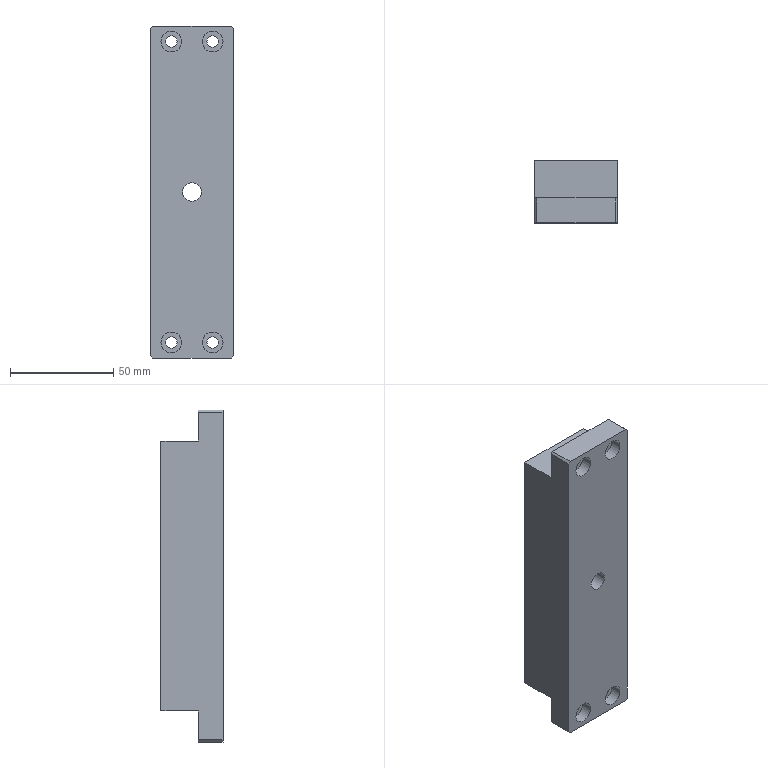Component | SolidWorks | XT-1-06-2-1 | 1 solid | 39 faces | box 40 x 30 x 160.5 mm | volume 165771 mm3 | cylinder 20 | plane 19 | commonest cylinder face diameters 10 x8 5.5 x8 15 x2 9 x2
build123d program:
from build123d import *

# Parameters (mm, degrees)
BOSS_EXTRUDE1_DEPTH                             = 40
M5_HEX_SOCKET_HEAD_CAP_SCREW_CBORE1_D           = 5.5
M5_HEX_SOCKET_HEAD_CAP_SCREW_CBORE1_CBORE_D     = 10
M5_HEX_SOCKET_HEAD_CAP_SCREW_CBORE1_CBORE_DEPTH = 5.4
M8_HEX_SOCKET_HEAD_CAP_SCREW_CBORE1_D           = 9
M8_HEX_SOCKET_HEAD_CAP_SCREW_CBORE1_CBORE_D     = 15
M8_HEX_SOCKET_HEAD_CAP_SCREW_CBORE1_CBORE_DEPTH = 8.6
CHAMFER1_SIZE                                   = 1


with BuildPart() as part:
    # Sketch1 → Boss-Extrude1 (new body)
    with BuildSketch(Plane.XY):
        Polygon((0, 0), (0, -12), (160.5, -12), (160.5, 0), (145.5, 0), (145.5, 18), (15, 18), (15, 0), align=None)
    extrude(amount=BOSS_EXTRUDE1_DEPTH)

    # M5 Hex Socket Head Cap Screw CBORE1 (through all)
    with Locations(Plane(origin=(0, -12, 0), x_dir=(-1, 0, 0), z_dir=(0, -1, 0))):
        with Locations((-7.5, -10), (-7.5, -30), (-153, -10), (-153, -30)):
            CounterBoreHole(M5_HEX_SOCKET_HEAD_CAP_SCREW_CBORE1_D / 2, M5_HEX_SOCKET_HEAD_CAP_SCREW_CBORE1_CBORE_D / 2, M5_HEX_SOCKET_HEAD_CAP_SCREW_CBORE1_CBORE_DEPTH)

    # M8 Hex Socket Head Cap Screw CBORE1 (through all)
    with Locations(Plane(origin=(0, 18, 0), x_dir=(1, 0, 0), z_dir=(0, 1, 0))):
        with Locations((80.25, -20)):
            CounterBoreHole(M8_HEX_SOCKET_HEAD_CAP_SCREW_CBORE1_D / 2, M8_HEX_SOCKET_HEAD_CAP_SCREW_CBORE1_CBORE_D / 2, M8_HEX_SOCKET_HEAD_CAP_SCREW_CBORE1_CBORE_DEPTH)

    # Chamfer1
    chamfer1_edges = [part.edges().sort_by_distance(p)[0] for p in [
        (0, -6, 0),
        (160.5, -6, 40),
        (0, -6, 40),
        (160.5, -6, 0),
    ]]
    chamfer(chamfer1_edges, length=CHAMFER1_SIZE)


solid = part.part

# Placed as in the assembly
solid = solid.moved(Location((884.283, 54.385, 7.5), (0, 90, 0)))